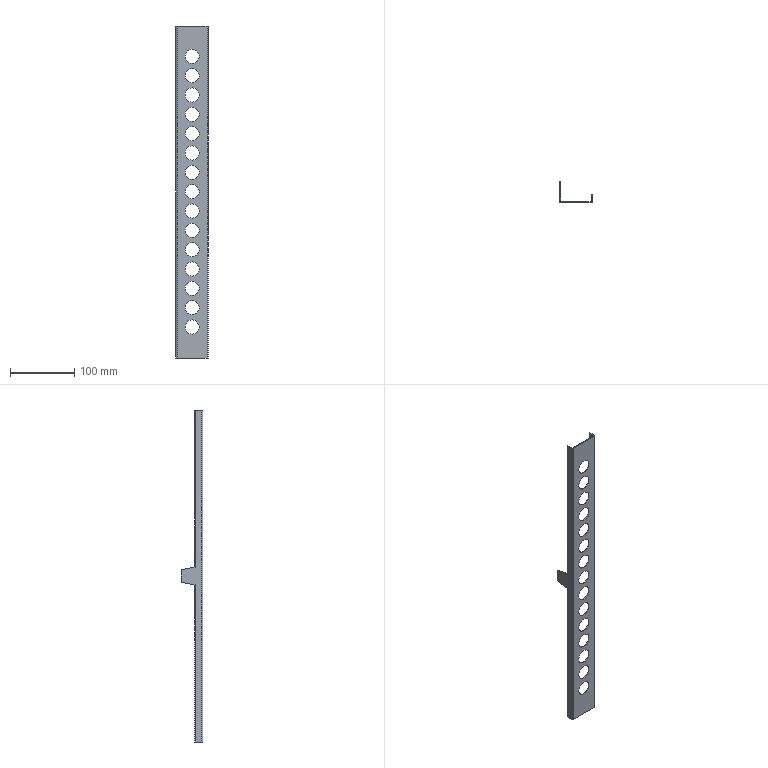Component | SolidWorks | RAY MONTAJ-1_tepsi _st dayama delikli-1 | 1 solid | 56 faces | volume 31336 mm3 | cylinder 34 | plane 22 | commonest cylinder face diameters 22 x30 3.473 x2 1.473 x2